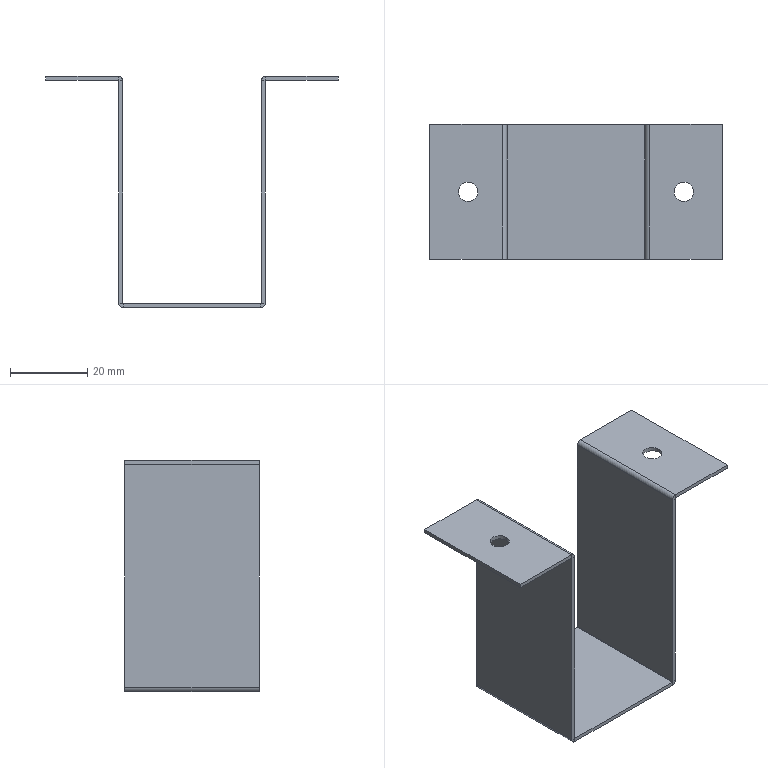Component | SolidWorks | CircuitBreakerBracket_2-1 | 1 solid | 42 faces | box 76 x 35 x 60 mm | volume 6715 mm3 | plane 30 | cylinder 12 | commonest cylinder face diameters 5 x4 2.2 x4 0.2 x4
STEP:
#1=COLOUR_RGB('',0.7922,0.8196,0.9333);
#2=FILL_AREA_STYLE_COLOUR('',#1);
#3=FILL_AREA_STYLE('',(#2));
#4=SURFACE_STYLE_FILL_AREA(#3);
#5=SURFACE_SIDE_STYLE('',(#4));
#6=SURFACE_STYLE_USAGE(.BOTH.,#5);
#7=PRESENTATION_STYLE_ASSIGNMENT((#6));
#8=CARTESIAN_POINT('',(1.068,-1.447,9.771));
#9=VERTEX_POINT('',#8);
#10=CARTESIAN_POINT('',(1.265,-1.447,9.771));
#11=VERTEX_POINT('',#10);
#12=CARTESIAN_POINT('',(1.167,-1.447,9.771));
#13=DIRECTION('',(0.,0.,1.));
#14=DIRECTION('',(1.,0.,0.));
#15=AXIS2_PLACEMENT_3D('',#12,#13,#14);
#16=CIRCLE('',#15,0.09843);
#17=EDGE_CURVE('',#9,#11,#16,.T.);
#18=ORIENTED_EDGE('',*,*,#17,.F.);
#19=CARTESIAN_POINT('',(1.068,-1.447,9.81));
#20=VERTEX_POINT('',#19);
#21=CARTESIAN_POINT('',(1.068,-1.447,9.771));
#22=DIRECTION('',(0.,0.,1.));
#23=VECTOR('',#22,39.37);
#24=LINE('',#21,#23);
#25=EDGE_CURVE('',#9,#20,#24,.T.);
#26=ORIENTED_EDGE('',*,*,#25,.T.);
#27=CARTESIAN_POINT('',(1.265,-1.447,9.81));
#28=VERTEX_POINT('',#27);
#29=CARTESIAN_POINT('',(1.167,-1.447,9.81));
#30=DIRECTION('',(0.,0.,1.));
#31=DIRECTION('',(1.,0.,0.));
#32=AXIS2_PLACEMENT_3D('',#29,#30,#31);
#33=CIRCLE('',#32,0.09843);
#34=EDGE_CURVE('',#20,#28,#33,.T.);
#35=ORIENTED_EDGE('',*,*,#34,.T.);
#36=CARTESIAN_POINT('',(1.265,-1.447,9.771));
#37=DIRECTION('',(0.,0.,1.));
#38=VECTOR('',#37,39.37);
#39=LINE('',#36,#38);
#40=EDGE_CURVE('',#11,#28,#39,.T.);
#41=ORIENTED_EDGE('',*,*,#40,.F.);
#42=EDGE_LOOP('',(#18,#26,#35,#41));
#43=FACE_OUTER_BOUND('',#42,.T.);
#44=CARTESIAN_POINT('',(1.167,-1.447,9.771));
#45=DIRECTION('',(0.,0.,1.));
#46=DIRECTION('',(1.,0.,0.));
#47=AXIS2_PLACEMENT_3D('',#44,#45,#46);
#48=CYLINDRICAL_SURFACE('',#47,0.09843);
#49=ADVANCED_FACE('',(#43),#48,.F.);
#50=CARTESIAN_POINT('',(-1.136,-1.447,9.771));
#51=VERTEX_POINT('',#50);
#52=CARTESIAN_POINT('',(-0.9394,-1.447,9.771));
#53=VERTEX_POINT('',#52);
#54=CARTESIAN_POINT('',(-1.038,-1.447,9.771));
#55=DIRECTION('',(0.,0.,1.));
#56=DIRECTION('',(1.,0.,0.));
#57=AXIS2_PLACEMENT_3D('',#54,#55,#56);
#58=CIRCLE('',#57,0.09843);
#59=EDGE_CURVE('',#51,#53,#58,.T.);
#60=ORIENTED_EDGE('',*,*,#59,.F.);
#61=CARTESIAN_POINT('',(-1.136,-1.447,9.81));
#62=VERTEX_POINT('',#61);
#63=CARTESIAN_POINT('',(-1.136,-1.447,9.771));
#64=DIRECTION('',(0.,0.,1.));
#65=VECTOR('',#64,39.37);
#66=LINE('',#63,#65);
#67=EDGE_CURVE('',#51,#62,#66,.T.);
#68=ORIENTED_EDGE('',*,*,#67,.T.);
#69=CARTESIAN_POINT('',(-0.9394,-1.447,9.81));
#70=VERTEX_POINT('',#69);
#71=CARTESIAN_POINT('',(-1.038,-1.447,9.81));
#72=DIRECTION('',(0.,0.,1.));
#73=DIRECTION('',(1.,0.,0.));
#74=AXIS2_PLACEMENT_3D('',#71,#72,#73);
#75=CIRCLE('',#74,0.09843);
#76=EDGE_CURVE('',#62,#70,#75,.T.);
#77=ORIENTED_EDGE('',*,*,#76,.T.);
#78=CARTESIAN_POINT('',(-0.9394,-1.447,9.771));
#79=DIRECTION('',(0.,0.,1.));
#80=VECTOR('',#79,39.37);
#81=LINE('',#78,#80);
#82=EDGE_CURVE('',#53,#70,#81,.T.);
#83=ORIENTED_EDGE('',*,*,#82,.F.);
#84=EDGE_LOOP('',(#60,#68,#77,#83));
#85=FACE_OUTER_BOUND('',#84,.T.);
#86=CARTESIAN_POINT('',(-1.038,-1.447,9.771));
#87=DIRECTION('',(0.,0.,1.));
#88=DIRECTION('',(1.,0.,0.));
#89=AXIS2_PLACEMENT_3D('',#86,#87,#88);
#90=CYLINDRICAL_SURFACE('',#89,0.09843);
#91=ADVANCED_FACE('',(#85),#90,.F.);
#92=CARTESIAN_POINT('',(0.8126,-2.136,9.767));
#93=VERTEX_POINT('',#92);
#94=CARTESIAN_POINT('',(0.7732,-2.136,9.767));
#95=VERTEX_POINT('',#94);
#96=CARTESIAN_POINT('',(0.8126,-2.136,9.767));
#97=DIRECTION('',(-1.,0.,0.));
#98=VECTOR('',#97,39.37);
#99=LINE('',#96,#98);
#100=EDGE_CURVE('',#93,#95,#99,.T.);
#101=ORIENTED_EDGE('',*,*,#100,.T.);
#102=CARTESIAN_POINT('',(0.7732,-2.136,7.491));
#103=VERTEX_POINT('',#102);
#104=CARTESIAN_POINT('',(0.7732,-2.136,7.488));
#105=DIRECTION('',(-0.,0.,-1.));
#106=VECTOR('',#105,39.37);
#107=LINE('',#104,#106);
#108=EDGE_CURVE('',#95,#103,#107,.T.);
#109=ORIENTED_EDGE('',*,*,#108,.T.);
#110=CARTESIAN_POINT('',(0.8126,-2.136,7.491));
#111=VERTEX_POINT('',#110);
#112=CARTESIAN_POINT('',(0.8126,-2.136,7.491));
#113=DIRECTION('',(1.,0.,-0.));
#114=VECTOR('',#113,39.37);
#115=LINE('',#112,#114);
#116=EDGE_CURVE('',#103,#111,#115,.T.);
#117=ORIENTED_EDGE('',*,*,#116,.T.);
#118=CARTESIAN_POINT('',(0.8126,-2.136,7.488));
#119=DIRECTION('',(-0.,0.,-1.));
#120=VECTOR('',#119,39.37);
#121=LINE('',#118,#120);
#122=EDGE_CURVE('',#93,#111,#121,.T.);
#123=ORIENTED_EDGE('',*,*,#122,.F.);
#124=EDGE_LOOP('',(#101,#109,#117,#123));
#125=FACE_OUTER_BOUND('',#124,.T.);
#126=CARTESIAN_POINT('',(0.8126,-2.136,7.488));
#127=DIRECTION('',(0.,1.,0.));
#128=DIRECTION('',(0.,0.,1.));
#129=AXIS2_PLACEMENT_3D('',#126,#127,#128);
#130=PLANE('',#129);
#131=ADVANCED_FACE('',(#125),#130,.F.);
#132=CARTESIAN_POINT('',(0.8126,-0.7579,9.767));
#133=VERTEX_POINT('',#132);
#134=CARTESIAN_POINT('',(0.7732,-0.7579,9.767));
#135=VERTEX_POINT('',#134);
#136=CARTESIAN_POINT('',(0.8126,-0.7579,9.767));
#137=DIRECTION('',(-1.,0.,0.));
#138=VECTOR('',#137,39.37);
#139=LINE('',#136,#138);
#140=EDGE_CURVE('',#133,#135,#139,.T.);
#141=ORIENTED_EDGE('',*,*,#140,.F.);
#142=CARTESIAN_POINT('',(0.8126,-0.7579,7.491));
#143=VERTEX_POINT('',#142);
#144=CARTESIAN_POINT('',(0.8126,-0.7579,7.488));
#145=DIRECTION('',(0.,0.,1.));
#146=VECTOR('',#145,39.37);
#147=LINE('',#144,#146);
#148=EDGE_CURVE('',#143,#133,#147,.T.);
#149=ORIENTED_EDGE('',*,*,#148,.F.);
#150=CARTESIAN_POINT('',(0.7732,-0.7579,7.491));
#151=VERTEX_POINT('',#150);
#152=CARTESIAN_POINT('',(0.7732,-0.7579,7.491));
#153=DIRECTION('',(1.,0.,-0.));
#154=VECTOR('',#153,39.37);
#155=LINE('',#152,#154);
#156=EDGE_CURVE('',#151,#143,#155,.T.);
#157=ORIENTED_EDGE('',*,*,#156,.F.);
#158=CARTESIAN_POINT('',(0.7732,-0.7579,9.81));
#159=DIRECTION('',(0.,0.,1.));
#160=VECTOR('',#159,39.37);
#161=LINE('',#158,#160);
#162=EDGE_CURVE('',#151,#135,#161,.T.);
#163=ORIENTED_EDGE('',*,*,#162,.T.);
#164=EDGE_LOOP('',(#141,#149,#157,#163));
#165=FACE_OUTER_BOUND('',#164,.T.);
#166=CARTESIAN_POINT('',(0.8126,-0.7579,9.81));
#167=DIRECTION('',(0.,-1.,0.));
#168=DIRECTION('',(0.,0.,-1.));
#169=AXIS2_PLACEMENT_3D('',#166,#167,#168);
#170=PLANE('',#169);
#171=ADVANCED_FACE('',(#165),#170,.F.);
#172=CARTESIAN_POINT('',(0.8126,-2.136,9.767));
#173=DIRECTION('',(0.,1.,0.));
#174=VECTOR('',#173,39.37);
#175=LINE('',#172,#174);
#176=EDGE_CURVE('',#93,#133,#175,.T.);
#177=ORIENTED_EDGE('',*,*,#176,.F.);
#178=ORIENTED_EDGE('',*,*,#122,.T.);
#179=CARTESIAN_POINT('',(0.8126,-2.136,7.491));
#180=DIRECTION('',(-0.,-1.,-0.));
#181=VECTOR('',#180,39.37);
#182=LINE('',#179,#181);
#183=EDGE_CURVE('',#143,#111,#182,.T.);
#184=ORIENTED_EDGE('',*,*,#183,.F.);
#185=ORIENTED_EDGE('',*,*,#148,.T.);
#186=EDGE_LOOP('',(#177,#178,#184,#185));
#187=FACE_OUTER_BOUND('',#186,.T.);
#188=CARTESIAN_POINT('',(0.8126,-2.275,7.488));
#189=DIRECTION('',(-1.,0.,0.));
#190=DIRECTION('',(0.,0.,1.));
#191=AXIS2_PLACEMENT_3D('',#188,#189,#190);
#192=PLANE('',#191);
#193=ADVANCED_FACE('',(#187),#192,.F.);
#194=ORIENTED_EDGE('',*,*,#108,.F.);
#195=CARTESIAN_POINT('',(0.7732,-2.136,9.767));
#196=DIRECTION('',(0.,1.,0.));
#197=VECTOR('',#196,39.37);
#198=LINE('',#195,#197);
#199=EDGE_CURVE('',#95,#135,#198,.T.);
#200=ORIENTED_EDGE('',*,*,#199,.T.);
#201=ORIENTED_EDGE('',*,*,#162,.F.);
#202=CARTESIAN_POINT('',(0.7732,-2.136,7.491));
#203=DIRECTION('',(0.,1.,0.));
#204=VECTOR('',#203,39.37);
#205=LINE('',#202,#204);
#206=EDGE_CURVE('',#103,#151,#205,.T.);
#207=ORIENTED_EDGE('',*,*,#206,.F.);
#208=EDGE_LOOP('',(#194,#200,#201,#207));
#209=FACE_OUTER_BOUND('',#208,.T.);
#210=CARTESIAN_POINT('',(0.7732,-2.275,7.488));
#211=DIRECTION('',(-1.,0.,0.));
#212=DIRECTION('',(0.,0.,1.));
#213=AXIS2_PLACEMENT_3D('',#210,#211,#212);
#214=PLANE('',#213);
#215=ADVANCED_FACE('',(#209),#214,.T.);
#216=CARTESIAN_POINT('',(-0.6835,-0.7579,9.767));
#217=VERTEX_POINT('',#216);
#218=CARTESIAN_POINT('',(-0.6441,-0.7579,9.767));
#219=VERTEX_POINT('',#218);
#220=CARTESIAN_POINT('',(-0.6835,-0.7579,9.767));
#221=DIRECTION('',(1.,0.,0.));
#222=VECTOR('',#221,39.37);
#223=LINE('',#220,#222);
#224=EDGE_CURVE('',#217,#219,#223,.T.);
#225=ORIENTED_EDGE('',*,*,#224,.T.);
#226=CARTESIAN_POINT('',(-0.6441,-0.7579,7.491));
#227=VERTEX_POINT('',#226);
#228=CARTESIAN_POINT('',(-0.6441,-0.7579,7.488));
#229=DIRECTION('',(0.,0.,-1.));
#230=VECTOR('',#229,39.37);
#231=LINE('',#228,#230);
#232=EDGE_CURVE('',#219,#227,#231,.T.);
#233=ORIENTED_EDGE('',*,*,#232,.T.);
#234=CARTESIAN_POINT('',(-0.6835,-0.7579,7.491));
#235=VERTEX_POINT('',#234);
#236=CARTESIAN_POINT('',(-0.6835,-0.7579,7.491));
#237=DIRECTION('',(-1.,0.,-0.));
#238=VECTOR('',#237,39.37);
#239=LINE('',#236,#238);
#240=EDGE_CURVE('',#227,#235,#239,.T.);
#241=ORIENTED_EDGE('',*,*,#240,.T.);
#242=CARTESIAN_POINT('',(-0.6835,-0.7579,7.488));
#243=DIRECTION('',(0.,0.,-1.));
#244=VECTOR('',#243,39.37);
#245=LINE('',#242,#244);
#246=EDGE_CURVE('',#217,#235,#245,.T.);
#247=ORIENTED_EDGE('',*,*,#246,.F.);
#248=EDGE_LOOP('',(#225,#233,#241,#247));
#249=FACE_OUTER_BOUND('',#248,.T.);
#250=CARTESIAN_POINT('',(-0.6835,-0.7579,7.488));
#251=DIRECTION('',(0.,-1.,0.));
#252=DIRECTION('',(0.,0.,-1.));
#253=AXIS2_PLACEMENT_3D('',#250,#251,#252);
#254=PLANE('',#253);
#255=ADVANCED_FACE('',(#249),#254,.F.);
#256=CARTESIAN_POINT('',(-0.6835,-2.136,9.767));
#257=VERTEX_POINT('',#256);
#258=CARTESIAN_POINT('',(-0.6441,-2.136,9.767));
#259=VERTEX_POINT('',#258);
#260=CARTESIAN_POINT('',(-0.6835,-2.136,9.767));
#261=DIRECTION('',(1.,0.,0.));
#262=VECTOR('',#261,39.37);
#263=LINE('',#260,#262);
#264=EDGE_CURVE('',#257,#259,#263,.T.);
#265=ORIENTED_EDGE('',*,*,#264,.F.);
#266=CARTESIAN_POINT('',(-0.6835,-2.136,7.491));
#267=VERTEX_POINT('',#266);
#268=CARTESIAN_POINT('',(-0.6835,-2.136,7.488));
#269=DIRECTION('',(-0.,0.,1.));
#270=VECTOR('',#269,39.37);
#271=LINE('',#268,#270);
#272=EDGE_CURVE('',#267,#257,#271,.T.);
#273=ORIENTED_EDGE('',*,*,#272,.F.);
#274=CARTESIAN_POINT('',(-0.6441,-2.136,7.491));
#275=VERTEX_POINT('',#274);
#276=CARTESIAN_POINT('',(-0.6441,-2.136,7.491));
#277=DIRECTION('',(-1.,0.,-0.));
#278=VECTOR('',#277,39.37);
#279=LINE('',#276,#278);
#280=EDGE_CURVE('',#275,#267,#279,.T.);
#281=ORIENTED_EDGE('',*,*,#280,.F.);
#282=CARTESIAN_POINT('',(-0.6441,-2.136,9.81));
#283=DIRECTION('',(-0.,0.,1.));
#284=VECTOR('',#283,39.37);
#285=LINE('',#282,#284);
#286=EDGE_CURVE('',#275,#259,#285,.T.);
#287=ORIENTED_EDGE('',*,*,#286,.T.);
#288=EDGE_LOOP('',(#265,#273,#281,#287));
#289=FACE_OUTER_BOUND('',#288,.T.);
#290=CARTESIAN_POINT('',(-0.6835,-2.136,9.81));
#291=DIRECTION('',(0.,1.,0.));
#292=DIRECTION('',(0.,0.,1.));
#293=AXIS2_PLACEMENT_3D('',#290,#291,#292);
#294=PLANE('',#293);
#295=ADVANCED_FACE('',(#289),#294,.F.);
#296=CARTESIAN_POINT('',(-0.6835,-0.7579,9.767));
#297=DIRECTION('',(0.,-1.,0.));
#298=VECTOR('',#297,39.37);
#299=LINE('',#296,#298);
#300=EDGE_CURVE('',#217,#257,#299,.T.);
#301=ORIENTED_EDGE('',*,*,#300,.F.);
#302=ORIENTED_EDGE('',*,*,#246,.T.);
#303=CARTESIAN_POINT('',(-0.6835,-0.7579,7.491));
#304=DIRECTION('',(0.,1.,0.));
#305=VECTOR('',#304,39.37);
#306=LINE('',#303,#305);
#307=EDGE_CURVE('',#267,#235,#306,.T.);
#308=ORIENTED_EDGE('',*,*,#307,.F.);
#309=ORIENTED_EDGE('',*,*,#272,.T.);
#310=EDGE_LOOP('',(#301,#302,#308,#309));
#311=FACE_OUTER_BOUND('',#310,.T.);
#312=CARTESIAN_POINT('',(-0.6835,-2.275,7.488));
#313=DIRECTION('',(1.,0.,0.));
#314=DIRECTION('',(0.,0.,-1.));
#315=AXIS2_PLACEMENT_3D('',#312,#313,#314);
#316=PLANE('',#315);
#317=ADVANCED_FACE('',(#311),#316,.F.);
#318=ORIENTED_EDGE('',*,*,#232,.F.);
#319=CARTESIAN_POINT('',(-0.6441,-0.7579,9.767));
#320=DIRECTION('',(0.,-1.,0.));
#321=VECTOR('',#320,39.37);
#322=LINE('',#319,#321);
#323=EDGE_CURVE('',#219,#259,#322,.T.);
#324=ORIENTED_EDGE('',*,*,#323,.T.);
#325=ORIENTED_EDGE('',*,*,#286,.F.);
#326=CARTESIAN_POINT('',(-0.6441,-0.7579,7.491));
#327=DIRECTION('',(0.,-1.,0.));
#328=VECTOR('',#327,39.37);
#329=LINE('',#326,#328);
#330=EDGE_CURVE('',#227,#275,#329,.T.);
#331=ORIENTED_EDGE('',*,*,#330,.F.);
#332=EDGE_LOOP('',(#318,#324,#325,#331));
#333=FACE_OUTER_BOUND('',#332,.T.);
#334=CARTESIAN_POINT('',(-0.6441,-2.275,7.488));
#335=DIRECTION('',(1.,0.,0.));
#336=DIRECTION('',(0.,0.,-1.));
#337=AXIS2_PLACEMENT_3D('',#334,#335,#336);
#338=PLANE('',#337);
#339=ADVANCED_FACE('',(#333),#338,.T.);
#340=CARTESIAN_POINT('',(0.7693,-0.7579,7.448));
#341=VERTEX_POINT('',#340);
#342=CARTESIAN_POINT('',(-0.6402,-0.7579,7.448));
#343=VERTEX_POINT('',#342);
#344=CARTESIAN_POINT('',(-0.6835,-0.7579,7.448));
#345=DIRECTION('',(-1.,0.,0.));
#346=VECTOR('',#345,39.37);
#347=LINE('',#344,#346);
#348=EDGE_CURVE('',#341,#343,#347,.T.);
#349=ORIENTED_EDGE('',*,*,#348,.F.);
#350=CARTESIAN_POINT('',(0.7693,-2.136,7.448));
#351=VERTEX_POINT('',#350);
#352=CARTESIAN_POINT('',(0.7693,-0.7579,7.448));
#353=DIRECTION('',(0.,-1.,0.));
#354=VECTOR('',#353,39.37);
#355=LINE('',#352,#354);
#356=EDGE_CURVE('',#341,#351,#355,.T.);
#357=ORIENTED_EDGE('',*,*,#356,.T.);
#358=CARTESIAN_POINT('',(-0.6402,-2.136,7.448));
#359=VERTEX_POINT('',#358);
#360=CARTESIAN_POINT('',(-0.6835,-2.136,7.448));
#361=DIRECTION('',(1.,0.,0.));
#362=VECTOR('',#361,39.37);
#363=LINE('',#360,#362);
#364=EDGE_CURVE('',#359,#351,#363,.T.);
#365=ORIENTED_EDGE('',*,*,#364,.F.);
#366=CARTESIAN_POINT('',(-0.6402,-2.136,7.448));
#367=DIRECTION('',(0.,1.,0.));
#368=VECTOR('',#367,39.37);
#369=LINE('',#366,#368);
#370=EDGE_CURVE('',#359,#343,#369,.T.);
#371=ORIENTED_EDGE('',*,*,#370,.T.);
#372=EDGE_LOOP('',(#349,#357,#365,#371));
#373=FACE_OUTER_BOUND('',#372,.T.);
#374=CARTESIAN_POINT('',(0.7651,-2.275,7.448));
#375=DIRECTION('',(0.,0.,-1.));
#376=DIRECTION('',(-1.,0.,0.));
#377=AXIS2_PLACEMENT_3D('',#374,#375,#376);
#378=PLANE('',#377);
#379=ADVANCED_FACE('',(#373),#378,.T.);
#380=CARTESIAN_POINT('',(0.7693,-0.7579,7.488));
#381=VERTEX_POINT('',#380);
#382=CARTESIAN_POINT('',(0.7693,-2.136,7.488));
#383=VERTEX_POINT('',#382);
#384=CARTESIAN_POINT('',(0.7693,-0.7579,7.488));
#385=DIRECTION('',(0.,-1.,0.));
#386=VECTOR('',#385,39.37);
#387=LINE('',#384,#386);
#388=EDGE_CURVE('',#381,#383,#387,.T.);
#389=ORIENTED_EDGE('',*,*,#388,.F.);
#390=CARTESIAN_POINT('',(-0.6402,-0.7579,7.488));
#391=VERTEX_POINT('',#390);
#392=CARTESIAN_POINT('',(-0.6835,-0.7579,7.488));
#393=DIRECTION('',(-1.,0.,0.));
#394=VECTOR('',#393,39.37);
#395=LINE('',#392,#394);
#396=EDGE_CURVE('',#381,#391,#395,.T.);
#397=ORIENTED_EDGE('',*,*,#396,.T.);
#398=CARTESIAN_POINT('',(-0.6402,-2.136,7.488));
#399=VERTEX_POINT('',#398);
#400=CARTESIAN_POINT('',(-0.6402,-2.136,7.488));
#401=DIRECTION('',(0.,1.,0.));
#402=VECTOR('',#401,39.37);
#403=LINE('',#400,#402);
#404=EDGE_CURVE('',#399,#391,#403,.T.);
#405=ORIENTED_EDGE('',*,*,#404,.F.);
#406=CARTESIAN_POINT('',(-0.6835,-2.136,7.488));
#407=DIRECTION('',(1.,0.,0.));
#408=VECTOR('',#407,39.37);
#409=LINE('',#406,#408);
#410=EDGE_CURVE('',#399,#383,#409,.T.);
#411=ORIENTED_EDGE('',*,*,#410,.T.);
#412=EDGE_LOOP('',(#389,#397,#405,#411));
#413=FACE_OUTER_BOUND('',#412,.T.);
#414=CARTESIAN_POINT('',(0.7651,-2.275,7.488));
#415=DIRECTION('',(0.,0.,-1.));
#416=DIRECTION('',(-1.,0.,0.));
#417=AXIS2_PLACEMENT_3D('',#414,#415,#416);
#418=PLANE('',#417);
#419=ADVANCED_FACE('',(#413),#418,.F.);
#420=ORIENTED_EDGE('',*,*,#396,.F.);
#421=CARTESIAN_POINT('',(0.7693,-0.7579,7.488));
#422=DIRECTION('',(0.,0.,-1.));
#423=VECTOR('',#422,39.37);
#424=LINE('',#421,#423);
#425=EDGE_CURVE('',#381,#341,#424,.T.);
#426=ORIENTED_EDGE('',*,*,#425,.T.);
#427=ORIENTED_EDGE('',*,*,#348,.T.);
#428=CARTESIAN_POINT('',(-0.6402,-0.7579,7.488));
#429=DIRECTION('',(0.,0.,-1.));
#430=VECTOR('',#429,39.37);
#431=LINE('',#428,#430);
#432=EDGE_CURVE('',#391,#343,#431,.T.);
#433=ORIENTED_EDGE('',*,*,#432,.F.);
#434=EDGE_LOOP('',(#420,#426,#427,#433));
#435=FACE_OUTER_BOUND('',#434,.T.);
#436=CARTESIAN_POINT('',(-0.6835,-0.7579,7.448));
#437=DIRECTION('',(0.,1.,0.));
#438=DIRECTION('',(0.,0.,1.));
#439=AXIS2_PLACEMENT_3D('',#436,#437,#438);
#440=PLANE('',#439);
#441=ADVANCED_FACE('',(#435),#440,.T.);
#442=CARTESIAN_POINT('',(0.7693,-2.136,7.488));
#443=DIRECTION('',(0.,0.,-1.));
#444=VECTOR('',#443,39.37);
#445=LINE('',#442,#444);
#446=EDGE_CURVE('',#383,#351,#445,.T.);
#447=ORIENTED_EDGE('',*,*,#446,.F.);
#448=ORIENTED_EDGE('',*,*,#410,.F.);
#449=CARTESIAN_POINT('',(-0.6402,-2.136,7.488));
#450=DIRECTION('',(0.,0.,-1.));
#451=VECTOR('',#450,39.37);
#452=LINE('',#449,#451);
#453=EDGE_CURVE('',#399,#359,#452,.T.);
#454=ORIENTED_EDGE('',*,*,#453,.T.);
#455=ORIENTED_EDGE('',*,*,#364,.T.);
#456=EDGE_LOOP('',(#447,#448,#454,#455));
#457=FACE_OUTER_BOUND('',#456,.T.);
#458=CARTESIAN_POINT('',(-0.6835,-2.136,7.448));
#459=DIRECTION('',(0.,-1.,0.));
#460=DIRECTION('',(0.,0.,-1.));
#461=AXIS2_PLACEMENT_3D('',#458,#459,#460);
#462=PLANE('',#461);
#463=ADVANCED_FACE('',(#457),#462,.T.);
#464=ORIENTED_EDGE('',*,*,#240,.F.);
#465=CARTESIAN_POINT('',(-0.6402,-0.7579,7.491));
#466=DIRECTION('',(0.,1.,0.));
#467=DIRECTION('',(0.,0.,-1.));
#468=AXIS2_PLACEMENT_3D('',#465,#466,#467);
#469=CIRCLE('',#468,0.003937);
#470=EDGE_CURVE('',#391,#227,#469,.T.);
#471=ORIENTED_EDGE('',*,*,#470,.F.);
#472=ORIENTED_EDGE('',*,*,#432,.T.);
#473=CARTESIAN_POINT('',(-0.6402,-0.7579,7.491));
#474=DIRECTION('',(0.,1.,0.));
#475=DIRECTION('',(0.,0.,-1.));
#476=AXIS2_PLACEMENT_3D('',#473,#474,#475);
#477=CIRCLE('',#476,0.04331);
#478=EDGE_CURVE('',#343,#235,#477,.T.);
#479=ORIENTED_EDGE('',*,*,#478,.T.);
#480=EDGE_LOOP('',(#464,#471,#472,#479));
#481=FACE_OUTER_BOUND('',#480,.T.);
#482=CARTESIAN_POINT('',(-0.6402,-0.7579,7.491));
#483=DIRECTION('',(0.,1.,0.));
#484=DIRECTION('',(0.,0.,1.));
#485=AXIS2_PLACEMENT_3D('',#482,#483,#484);
#486=PLANE('',#485);
#487=ADVANCED_FACE('',(#481),#486,.T.);
#488=CARTESIAN_POINT('',(-0.6402,-2.136,7.491));
#489=DIRECTION('',(0.,-1.,0.));
#490=DIRECTION('',(0.,0.,-1.));
#491=AXIS2_PLACEMENT_3D('',#488,#489,#490);
#492=CIRCLE('',#491,0.003937);
#493=EDGE_CURVE('',#275,#399,#492,.T.);
#494=ORIENTED_EDGE('',*,*,#493,.F.);
#495=ORIENTED_EDGE('',*,*,#280,.T.);
#496=CARTESIAN_POINT('',(-0.6402,-2.136,7.491));
#497=DIRECTION('',(0.,-1.,0.));
#498=DIRECTION('',(0.,0.,-1.));
#499=AXIS2_PLACEMENT_3D('',#496,#497,#498);
#500=CIRCLE('',#499,0.04331);
#501=EDGE_CURVE('',#267,#359,#500,.T.);
#502=ORIENTED_EDGE('',*,*,#501,.T.);
#503=ORIENTED_EDGE('',*,*,#453,.F.);
#504=EDGE_LOOP('',(#494,#495,#502,#503));
#505=FACE_OUTER_BOUND('',#504,.T.);
#506=CARTESIAN_POINT('',(-0.6402,-2.136,7.491));
#507=DIRECTION('',(0.,1.,0.));
#508=DIRECTION('',(0.,0.,1.));
#509=AXIS2_PLACEMENT_3D('',#506,#507,#508);
#510=PLANE('',#509);
#511=ADVANCED_FACE('',(#505),#510,.F.);
#512=ORIENTED_EDGE('',*,*,#370,.F.);
#513=ORIENTED_EDGE('',*,*,#501,.F.);
#514=ORIENTED_EDGE('',*,*,#307,.T.);
#515=ORIENTED_EDGE('',*,*,#478,.F.);
#516=EDGE_LOOP('',(#512,#513,#514,#515));
#517=FACE_OUTER_BOUND('',#516,.T.);
#518=CARTESIAN_POINT('',(-0.6402,-2.136,7.491));
#519=DIRECTION('',(0.,-1.,0.));
#520=DIRECTION('',(-1.,0.,0.));
#521=AXIS2_PLACEMENT_3D('',#518,#519,#520);
#522=CYLINDRICAL_SURFACE('',#521,0.04331);
#523=ADVANCED_FACE('',(#517),#522,.T.);
#524=ORIENTED_EDGE('',*,*,#404,.T.);
#525=ORIENTED_EDGE('',*,*,#470,.T.);
#526=ORIENTED_EDGE('',*,*,#330,.T.);
#527=ORIENTED_EDGE('',*,*,#493,.T.);
#528=EDGE_LOOP('',(#524,#525,#526,#527));
#529=FACE_OUTER_BOUND('',#528,.T.);
#530=CARTESIAN_POINT('',(-0.6402,-2.136,7.491));
#531=DIRECTION('',(0.,-1.,0.));
#532=DIRECTION('',(-1.,0.,0.));
#533=AXIS2_PLACEMENT_3D('',#530,#531,#532);
#534=CYLINDRICAL_SURFACE('',#533,0.003937);
#535=ADVANCED_FACE('',(#529),#534,.F.);
#536=ORIENTED_EDGE('',*,*,#116,.F.);
#537=CARTESIAN_POINT('',(0.7693,-2.136,7.491));
#538=DIRECTION('',(0.,-1.,0.));
#539=DIRECTION('',(-1.,0.,0.));
#540=AXIS2_PLACEMENT_3D('',#537,#538,#539);
#541=CIRCLE('',#540,0.003937);
#542=EDGE_CURVE('',#383,#103,#541,.T.);
#543=ORIENTED_EDGE('',*,*,#542,.F.);
#544=ORIENTED_EDGE('',*,*,#446,.T.);
#545=CARTESIAN_POINT('',(0.7693,-2.136,7.491));
#546=DIRECTION('',(0.,-1.,0.));
#547=DIRECTION('',(-1.,0.,0.));
#548=AXIS2_PLACEMENT_3D('',#545,#546,#547);
#549=CIRCLE('',#548,0.04331);
#550=EDGE_CURVE('',#351,#111,#549,.T.);
#551=ORIENTED_EDGE('',*,*,#550,.T.);
#552=EDGE_LOOP('',(#536,#543,#544,#551));
#553=FACE_OUTER_BOUND('',#552,.T.);
#554=CARTESIAN_POINT('',(0.7693,-2.136,7.491));
#555=DIRECTION('',(0.,-1.,0.));
#556=DIRECTION('',(1.,0.,0.));
#557=AXIS2_PLACEMENT_3D('',#554,#555,#556);
#558=PLANE('',#557);
#559=ADVANCED_FACE('',(#553),#558,.T.);
#560=CARTESIAN_POINT('',(0.7693,-0.7579,7.491));
#561=DIRECTION('',(-0.,1.,0.));
#562=DIRECTION('',(-1.,0.,0.));
#563=AXIS2_PLACEMENT_3D('',#560,#561,#562);
#564=CIRCLE('',#563,0.003937);
#565=EDGE_CURVE('',#151,#381,#564,.T.);
#566=ORIENTED_EDGE('',*,*,#565,.F.);
#567=ORIENTED_EDGE('',*,*,#156,.T.);
#568=CARTESIAN_POINT('',(0.7693,-0.7579,7.491));
#569=DIRECTION('',(-0.,1.,0.));
#570=DIRECTION('',(-1.,0.,0.));
#571=AXIS2_PLACEMENT_3D('',#568,#569,#570);
#572=CIRCLE('',#571,0.04331);
#573=EDGE_CURVE('',#143,#341,#572,.T.);
#574=ORIENTED_EDGE('',*,*,#573,.T.);
#575=ORIENTED_EDGE('',*,*,#425,.F.);
#576=EDGE_LOOP('',(#566,#567,#574,#575));
#577=FACE_OUTER_BOUND('',#576,.T.);
#578=CARTESIAN_POINT('',(0.7693,-0.7579,7.491));
#579=DIRECTION('',(0.,-1.,0.));
#580=DIRECTION('',(1.,0.,0.));
#581=AXIS2_PLACEMENT_3D('',#578,#579,#580);
#582=PLANE('',#581);
#583=ADVANCED_FACE('',(#577),#582,.F.);
#584=ORIENTED_EDGE('',*,*,#356,.F.);
#585=ORIENTED_EDGE('',*,*,#573,.F.);
#586=ORIENTED_EDGE('',*,*,#183,.T.);
#587=ORIENTED_EDGE('',*,*,#550,.F.);
#588=EDGE_LOOP('',(#584,#585,#586,#587));
#589=FACE_OUTER_BOUND('',#588,.T.);
#590=CARTESIAN_POINT('',(0.7693,-0.7579,7.491));
#591=DIRECTION('',(-0.,1.,0.));
#592=DIRECTION('',(1.,0.,0.));
#593=AXIS2_PLACEMENT_3D('',#590,#591,#592);
#594=CYLINDRICAL_SURFACE('',#593,0.04331);
#595=ADVANCED_FACE('',(#589),#594,.T.);
#596=ORIENTED_EDGE('',*,*,#388,.T.);
#597=ORIENTED_EDGE('',*,*,#542,.T.);
#598=ORIENTED_EDGE('',*,*,#206,.T.);
#599=ORIENTED_EDGE('',*,*,#565,.T.);
#600=EDGE_LOOP('',(#596,#597,#598,#599));
#601=FACE_OUTER_BOUND('',#600,.T.);
#602=CARTESIAN_POINT('',(0.7693,-0.7579,7.491));
#603=DIRECTION('',(-0.,1.,0.));
#604=DIRECTION('',(1.,0.,0.));
#605=AXIS2_PLACEMENT_3D('',#602,#603,#604);
#606=CYLINDRICAL_SURFACE('',#605,0.003937);
#607=ADVANCED_FACE('',(#601),#606,.F.);
#608=CARTESIAN_POINT('',(-0.6874,-2.136,9.771));
#609=VERTEX_POINT('',#608);
#610=CARTESIAN_POINT('',(-0.6874,-2.136,9.81));
#611=VERTEX_POINT('',#610);
#612=CARTESIAN_POINT('',(-0.6874,-2.136,9.81));
#613=DIRECTION('',(0.,0.,1.));
#614=VECTOR('',#613,39.37);
#615=LINE('',#612,#614);
#616=EDGE_CURVE('',#609,#611,#615,.T.);
#617=ORIENTED_EDGE('',*,*,#616,.F.);
#618=CARTESIAN_POINT('',(-0.6874,-2.136,9.767));
#619=DIRECTION('',(0.,-1.,0.));
#620=DIRECTION('',(0.,0.,1.));
#621=AXIS2_PLACEMENT_3D('',#618,#619,#620);
#622=CIRCLE('',#621,0.003937);
#623=EDGE_CURVE('',#257,#609,#622,.T.);
#624=ORIENTED_EDGE('',*,*,#623,.F.);
#625=ORIENTED_EDGE('',*,*,#264,.T.);
#626=CARTESIAN_POINT('',(-0.6874,-2.136,9.767));
#627=DIRECTION('',(0.,-1.,0.));
#628=DIRECTION('',(0.,0.,1.));
#629=AXIS2_PLACEMENT_3D('',#626,#627,#628);
#630=CIRCLE('',#629,0.04331);
#631=EDGE_CURVE('',#259,#611,#630,.T.);
#632=ORIENTED_EDGE('',*,*,#631,.T.);
#633=EDGE_LOOP('',(#617,#624,#625,#632));
#634=FACE_OUTER_BOUND('',#633,.T.);
#635=CARTESIAN_POINT('',(-0.6874,-2.136,9.767));
#636=DIRECTION('',(0.,-1.,0.));
#637=DIRECTION('',(0.,0.,-1.));
#638=AXIS2_PLACEMENT_3D('',#635,#636,#637);
#639=PLANE('',#638);
#640=ADVANCED_FACE('',(#634),#639,.T.);
#641=CARTESIAN_POINT('',(-0.6874,-0.7579,9.771));
#642=VERTEX_POINT('',#641);
#643=CARTESIAN_POINT('',(-0.6874,-0.7579,9.767));
#644=DIRECTION('',(0.,1.,0.));
#645=DIRECTION('',(0.,0.,1.));
#646=AXIS2_PLACEMENT_3D('',#643,#644,#645);
#647=CIRCLE('',#646,0.003937);
#648=EDGE_CURVE('',#642,#217,#647,.T.);
#649=ORIENTED_EDGE('',*,*,#648,.F.);
#650=CARTESIAN_POINT('',(-0.6874,-0.7579,9.81));
#651=VERTEX_POINT('',#650);
#652=CARTESIAN_POINT('',(-0.6874,-0.7579,9.771));
#653=DIRECTION('',(0.,0.,1.));
#654=VECTOR('',#653,39.37);
#655=LINE('',#652,#654);
#656=EDGE_CURVE('',#642,#651,#655,.T.);
#657=ORIENTED_EDGE('',*,*,#656,.T.);
#658=CARTESIAN_POINT('',(-0.6874,-0.7579,9.767));
#659=DIRECTION('',(0.,1.,0.));
#660=DIRECTION('',(0.,0.,1.));
#661=AXIS2_PLACEMENT_3D('',#658,#659,#660);
#662=CIRCLE('',#661,0.04331);
#663=EDGE_CURVE('',#651,#219,#662,.T.);
#664=ORIENTED_EDGE('',*,*,#663,.T.);
#665=ORIENTED_EDGE('',*,*,#224,.F.);
#666=EDGE_LOOP('',(#649,#657,#664,#665));
#667=FACE_OUTER_BOUND('',#666,.T.);
#668=CARTESIAN_POINT('',(-0.6874,-0.7579,9.767));
#669=DIRECTION('',(0.,-1.,0.));
#670=DIRECTION('',(0.,0.,-1.));
#671=AXIS2_PLACEMENT_3D('',#668,#669,#670);
#672=PLANE('',#671);
#673=ADVANCED_FACE('',(#667),#672,.F.);
#674=ORIENTED_EDGE('',*,*,#323,.F.);
#675=ORIENTED_EDGE('',*,*,#663,.F.);
#676=CARTESIAN_POINT('',(-0.6874,-2.275,9.81));
#677=DIRECTION('',(0.,1.,0.));
#678=VECTOR('',#677,39.37);
#679=LINE('',#676,#678);
#680=EDGE_CURVE('',#611,#651,#679,.T.);
#681=ORIENTED_EDGE('',*,*,#680,.F.);
#682=ORIENTED_EDGE('',*,*,#631,.F.);
#683=EDGE_LOOP('',(#674,#675,#681,#682));
#684=FACE_OUTER_BOUND('',#683,.T.);
#685=CARTESIAN_POINT('',(-0.6874,-0.7579,9.767));
#686=DIRECTION('',(0.,1.,0.));
#687=DIRECTION('',(0.,0.,1.));
#688=AXIS2_PLACEMENT_3D('',#685,#686,#687);
#689=CYLINDRICAL_SURFACE('',#688,0.04331);
#690=ADVANCED_FACE('',(#684),#689,.T.);
#691=ORIENTED_EDGE('',*,*,#300,.T.);
#692=ORIENTED_EDGE('',*,*,#623,.T.);
#693=CARTESIAN_POINT('',(-0.6874,-2.136,9.771));
#694=DIRECTION('',(0.,1.,0.));
#695=VECTOR('',#694,39.37);
#696=LINE('',#693,#695);
#697=EDGE_CURVE('',#609,#642,#696,.T.);
#698=ORIENTED_EDGE('',*,*,#697,.T.);
#699=ORIENTED_EDGE('',*,*,#648,.T.);
#700=EDGE_LOOP('',(#691,#692,#698,#699));
#701=FACE_OUTER_BOUND('',#700,.T.);
#702=CARTESIAN_POINT('',(-0.6874,-0.7579,9.767));
#703=DIRECTION('',(0.,1.,0.));
#704=DIRECTION('',(0.,0.,1.));
#705=AXIS2_PLACEMENT_3D('',#702,#703,#704);
#706=CYLINDRICAL_SURFACE('',#705,0.003937);
#707=ADVANCED_FACE('',(#701),#706,.F.);
#708=CARTESIAN_POINT('',(-1.432,-0.7579,9.81));
#709=VERTEX_POINT('',#708);
#710=CARTESIAN_POINT('',(-0.6835,-0.7579,9.81));
#711=DIRECTION('',(1.,0.,0.));
#712=VECTOR('',#711,39.37);
#713=LINE('',#710,#712);
#714=EDGE_CURVE('',#709,#651,#713,.T.);
#715=ORIENTED_EDGE('',*,*,#714,.T.);
#716=ORIENTED_EDGE('',*,*,#656,.F.);
#717=CARTESIAN_POINT('',(-1.432,-0.7579,9.771));
#718=VERTEX_POINT('',#717);
#719=CARTESIAN_POINT('',(0.7651,-0.7579,9.771));
#720=DIRECTION('',(1.,0.,0.));
#721=VECTOR('',#720,39.37);
#722=LINE('',#719,#721);
#723=EDGE_CURVE('',#718,#642,#722,.T.);
#724=ORIENTED_EDGE('',*,*,#723,.F.);
#725=CARTESIAN_POINT('',(-1.432,-0.7579,9.81));
#726=DIRECTION('',(0.,0.,-1.));
#727=VECTOR('',#726,39.37);
#728=LINE('',#725,#727);
#729=EDGE_CURVE('',#709,#718,#728,.T.);
#730=ORIENTED_EDGE('',*,*,#729,.F.);
#731=EDGE_LOOP('',(#715,#716,#724,#730));
#732=FACE_OUTER_BOUND('',#731,.T.);
#733=CARTESIAN_POINT('',(-0.6835,-0.7579,9.81));
#734=DIRECTION('',(0.,1.,0.));
#735=DIRECTION('',(0.,0.,1.));
#736=AXIS2_PLACEMENT_3D('',#733,#734,#735);
#737=PLANE('',#736);
#738=ADVANCED_FACE('',(#732),#737,.T.);
#739=CARTESIAN_POINT('',(-1.432,-2.136,9.771));
#740=VERTEX_POINT('',#739);
#741=CARTESIAN_POINT('',(0.7651,-2.136,9.771));
#742=DIRECTION('',(-1.,0.,0.));
#743=VECTOR('',#742,39.37);
#744=LINE('',#741,#743);
#745=EDGE_CURVE('',#609,#740,#744,.T.);
#746=ORIENTED_EDGE('',*,*,#745,.F.);
#747=ORIENTED_EDGE('',*,*,#616,.T.);
#748=CARTESIAN_POINT('',(-1.432,-2.136,9.81));
#749=VERTEX_POINT('',#748);
#750=CARTESIAN_POINT('',(-1.432,-2.136,9.81));
#751=DIRECTION('',(-1.,0.,0.));
#752=VECTOR('',#751,39.37);
#753=LINE('',#750,#752);
#754=EDGE_CURVE('',#611,#749,#753,.T.);
#755=ORIENTED_EDGE('',*,*,#754,.T.);
#756=CARTESIAN_POINT('',(-1.432,-2.136,9.81));
#757=DIRECTION('',(0.,0.,-1.));
#758=VECTOR('',#757,39.37);
#759=LINE('',#756,#758);
#760=EDGE_CURVE('',#749,#740,#759,.T.);
#761=ORIENTED_EDGE('',*,*,#760,.T.);
#762=EDGE_LOOP('',(#746,#747,#755,#761));
#763=FACE_OUTER_BOUND('',#762,.T.);
#764=CARTESIAN_POINT('',(-1.432,-2.136,9.81));
#765=DIRECTION('',(0.,-1.,0.));
#766=DIRECTION('',(0.,0.,-1.));
#767=AXIS2_PLACEMENT_3D('',#764,#765,#766);
#768=PLANE('',#767);
#769=ADVANCED_FACE('',(#763),#768,.T.);
#770=CARTESIAN_POINT('',(-1.038,-1.447,9.81));
#771=DIRECTION('',(0.,0.,1.));
#772=DIRECTION('',(1.,0.,0.));
#773=AXIS2_PLACEMENT_3D('',#770,#771,#772);
#774=CIRCLE('',#773,0.09843);
#775=EDGE_CURVE('',#70,#62,#774,.T.);
#776=ORIENTED_EDGE('',*,*,#775,.F.);
#777=ORIENTED_EDGE('',*,*,#76,.F.);
#778=EDGE_LOOP('',(#776,#777));
#779=FACE_BOUND('',#778,.T.);
#780=ORIENTED_EDGE('',*,*,#754,.F.);
#781=ORIENTED_EDGE('',*,*,#680,.T.);
#782=ORIENTED_EDGE('',*,*,#714,.F.);
#783=CARTESIAN_POINT('',(-1.432,-0.7579,9.81));
#784=DIRECTION('',(0.,1.,0.));
#785=VECTOR('',#784,39.37);
#786=LINE('',#783,#785);
#787=EDGE_CURVE('',#749,#709,#786,.T.);
#788=ORIENTED_EDGE('',*,*,#787,.F.);
#789=EDGE_LOOP('',(#780,#781,#782,#788));
#790=FACE_OUTER_BOUND('',#789,.T.);
#791=CARTESIAN_POINT('',(0.7651,-2.275,9.81));
#792=DIRECTION('',(0.,0.,1.));
#793=DIRECTION('',(1.,0.,0.));
#794=AXIS2_PLACEMENT_3D('',#791,#792,#793);
#795=PLANE('',#794);
#796=ADVANCED_FACE('',(#779,#790),#795,.T.);
#797=CARTESIAN_POINT('',(-1.038,-1.447,9.771));
#798=DIRECTION('',(0.,0.,1.));
#799=DIRECTION('',(1.,0.,0.));
#800=AXIS2_PLACEMENT_3D('',#797,#798,#799);
#801=CIRCLE('',#800,0.09843);
#802=EDGE_CURVE('',#53,#51,#801,.T.);
#803=ORIENTED_EDGE('',*,*,#802,.T.);
#804=ORIENTED_EDGE('',*,*,#59,.T.);
#805=EDGE_LOOP('',(#803,#804));
#806=FACE_BOUND('',#805,.T.);
#807=ORIENTED_EDGE('',*,*,#697,.F.);
#808=ORIENTED_EDGE('',*,*,#745,.T.);
#809=CARTESIAN_POINT('',(-1.432,-2.275,9.771));
#810=DIRECTION('',(0.,1.,0.));
#811=VECTOR('',#810,39.37);
#812=LINE('',#809,#811);
#813=EDGE_CURVE('',#740,#718,#812,.T.);
#814=ORIENTED_EDGE('',*,*,#813,.T.);
#815=ORIENTED_EDGE('',*,*,#723,.T.);
#816=EDGE_LOOP('',(#807,#808,#814,#815));
#817=FACE_OUTER_BOUND('',#816,.T.);
#818=CARTESIAN_POINT('',(0.7651,-2.275,9.771));
#819=DIRECTION('',(0.,0.,1.));
#820=DIRECTION('',(1.,0.,0.));
#821=AXIS2_PLACEMENT_3D('',#818,#819,#820);
#822=PLANE('',#821);
#823=ADVANCED_FACE('',(#806,#817),#822,.F.);
#824=ORIENTED_EDGE('',*,*,#813,.F.);
#825=ORIENTED_EDGE('',*,*,#760,.F.);
#826=ORIENTED_EDGE('',*,*,#787,.T.);
#827=ORIENTED_EDGE('',*,*,#729,.T.);
#828=EDGE_LOOP('',(#824,#825,#826,#827));
#829=FACE_OUTER_BOUND('',#828,.T.);
#830=CARTESIAN_POINT('',(-1.432,-0.7579,9.81));
#831=DIRECTION('',(-1.,0.,-0.));
#832=DIRECTION('',(-0.,0.,1.));
#833=AXIS2_PLACEMENT_3D('',#830,#831,#832);
#834=PLANE('',#833);
#835=ADVANCED_FACE('',(#829),#834,.T.);
#836=CARTESIAN_POINT('',(0.8165,-0.7579,9.771));
#837=VERTEX_POINT('',#836);
#838=CARTESIAN_POINT('',(0.8165,-0.7579,9.81));
#839=VERTEX_POINT('',#838);
#840=CARTESIAN_POINT('',(0.8165,-0.7579,9.81));
#841=DIRECTION('',(0.,0.,1.));
#842=VECTOR('',#841,39.37);
#843=LINE('',#840,#842);
#844=EDGE_CURVE('',#837,#839,#843,.T.);
#845=ORIENTED_EDGE('',*,*,#844,.F.);
#846=CARTESIAN_POINT('',(0.8165,-0.7579,9.767));
#847=DIRECTION('',(0.,1.,0.));
#848=DIRECTION('',(0.,0.,-1.));
#849=AXIS2_PLACEMENT_3D('',#846,#847,#848);
#850=CIRCLE('',#849,0.003937);
#851=EDGE_CURVE('',#133,#837,#850,.T.);
#852=ORIENTED_EDGE('',*,*,#851,.F.);
#853=ORIENTED_EDGE('',*,*,#140,.T.);
#854=CARTESIAN_POINT('',(0.8165,-0.7579,9.767));
#855=DIRECTION('',(0.,1.,0.));
#856=DIRECTION('',(0.,0.,-1.));
#857=AXIS2_PLACEMENT_3D('',#854,#855,#856);
#858=CIRCLE('',#857,0.04331);
#859=EDGE_CURVE('',#135,#839,#858,.T.);
#860=ORIENTED_EDGE('',*,*,#859,.T.);
#861=EDGE_LOOP('',(#845,#852,#853,#860));
#862=FACE_OUTER_BOUND('',#861,.T.);
#863=CARTESIAN_POINT('',(0.8165,-0.7579,9.767));
#864=DIRECTION('',(0.,1.,0.));
#865=DIRECTION('',(0.,0.,1.));
#866=AXIS2_PLACEMENT_3D('',#863,#864,#865);
#867=PLANE('',#866);
#868=ADVANCED_FACE('',(#862),#867,.T.);
#869=CARTESIAN_POINT('',(0.8165,-2.136,9.771));
#870=VERTEX_POINT('',#869);
#871=CARTESIAN_POINT('',(0.8165,-2.136,9.767));
#872=DIRECTION('',(0.,-1.,0.));
#873=DIRECTION('',(0.,0.,-1.));
#874=AXIS2_PLACEMENT_3D('',#871,#872,#873);
#875=CIRCLE('',#874,0.003937);
#876=EDGE_CURVE('',#870,#93,#875,.T.);
#877=ORIENTED_EDGE('',*,*,#876,.F.);
#878=CARTESIAN_POINT('',(0.8165,-2.136,9.81));
#879=VERTEX_POINT('',#878);
#880=CARTESIAN_POINT('',(0.8165,-2.136,9.771));
#881=DIRECTION('',(0.,0.,1.));
#882=VECTOR('',#881,39.37);
#883=LINE('',#880,#882);
#884=EDGE_CURVE('',#870,#879,#883,.T.);
#885=ORIENTED_EDGE('',*,*,#884,.T.);
#886=CARTESIAN_POINT('',(0.8165,-2.136,9.767));
#887=DIRECTION('',(0.,-1.,0.));
#888=DIRECTION('',(0.,0.,-1.));
#889=AXIS2_PLACEMENT_3D('',#886,#887,#888);
#890=CIRCLE('',#889,0.04331);
#891=EDGE_CURVE('',#879,#95,#890,.T.);
#892=ORIENTED_EDGE('',*,*,#891,.T.);
#893=ORIENTED_EDGE('',*,*,#100,.F.);
#894=EDGE_LOOP('',(#877,#885,#892,#893));
#895=FACE_OUTER_BOUND('',#894,.T.);
#896=CARTESIAN_POINT('',(0.8165,-2.136,9.767));
#897=DIRECTION('',(0.,1.,0.));
#898=DIRECTION('',(0.,0.,1.));
#899=AXIS2_PLACEMENT_3D('',#896,#897,#898);
#900=PLANE('',#899);
#901=ADVANCED_FACE('',(#895),#900,.F.);
#902=ORIENTED_EDGE('',*,*,#199,.F.);
#903=ORIENTED_EDGE('',*,*,#891,.F.);
#904=CARTESIAN_POINT('',(0.8165,-0.7579,9.81));
#905=DIRECTION('',(0.,1.,0.));
#906=VECTOR('',#905,39.37);
#907=LINE('',#904,#906);
#908=EDGE_CURVE('',#879,#839,#907,.T.);
#909=ORIENTED_EDGE('',*,*,#908,.T.);
#910=ORIENTED_EDGE('',*,*,#859,.F.);
#911=EDGE_LOOP('',(#902,#903,#909,#910));
#912=FACE_OUTER_BOUND('',#911,.T.);
#913=CARTESIAN_POINT('',(0.8165,-2.136,9.767));
#914=DIRECTION('',(0.,-1.,0.));
#915=DIRECTION('',(0.,0.,1.));
#916=AXIS2_PLACEMENT_3D('',#913,#914,#915);
#917=CYLINDRICAL_SURFACE('',#916,0.04331);
#918=ADVANCED_FACE('',(#912),#917,.T.);
#919=ORIENTED_EDGE('',*,*,#176,.T.);
#920=ORIENTED_EDGE('',*,*,#851,.T.);
#921=CARTESIAN_POINT('',(0.8165,-0.7579,9.771));
#922=DIRECTION('',(0.,-1.,0.));
#923=VECTOR('',#922,39.37);
#924=LINE('',#921,#923);
#925=EDGE_CURVE('',#837,#870,#924,.T.);
#926=ORIENTED_EDGE('',*,*,#925,.T.);
#927=ORIENTED_EDGE('',*,*,#876,.T.);
#928=EDGE_LOOP('',(#919,#920,#926,#927));
#929=FACE_OUTER_BOUND('',#928,.T.);
#930=CARTESIAN_POINT('',(0.8165,-2.136,9.767));
#931=DIRECTION('',(0.,-1.,0.));
#932=DIRECTION('',(0.,0.,1.));
#933=AXIS2_PLACEMENT_3D('',#930,#931,#932);
#934=CYLINDRICAL_SURFACE('',#933,0.003937);
#935=ADVANCED_FACE('',(#929),#934,.F.);
#936=CARTESIAN_POINT('',(1.561,-0.7579,9.771));
#937=VERTEX_POINT('',#936);
#938=CARTESIAN_POINT('',(0.7651,-0.7579,9.771));
#939=DIRECTION('',(1.,0.,0.));
#940=VECTOR('',#939,39.37);
#941=LINE('',#938,#940);
#942=EDGE_CURVE('',#837,#937,#941,.T.);
#943=ORIENTED_EDGE('',*,*,#942,.F.);
#944=ORIENTED_EDGE('',*,*,#844,.T.);
#945=CARTESIAN_POINT('',(1.561,-0.7579,9.81));
#946=VERTEX_POINT('',#945);
#947=CARTESIAN_POINT('',(0.8126,-0.7579,9.81));
#948=DIRECTION('',(1.,0.,0.));
#949=VECTOR('',#948,39.37);
#950=LINE('',#947,#949);
#951=EDGE_CURVE('',#839,#946,#950,.T.);
#952=ORIENTED_EDGE('',*,*,#951,.T.);
#953=CARTESIAN_POINT('',(1.561,-0.7579,9.81));
#954=DIRECTION('',(-0.,0.,-1.));
#955=VECTOR('',#954,39.37);
#956=LINE('',#953,#955);
#957=EDGE_CURVE('',#946,#937,#956,.T.);
#958=ORIENTED_EDGE('',*,*,#957,.T.);
#959=EDGE_LOOP('',(#943,#944,#952,#958));
#960=FACE_OUTER_BOUND('',#959,.T.);
#961=CARTESIAN_POINT('',(0.8126,-0.7579,9.81));
#962=DIRECTION('',(0.,1.,0.));
#963=DIRECTION('',(0.,0.,1.));
#964=AXIS2_PLACEMENT_3D('',#961,#962,#963);
#965=PLANE('',#964);
#966=ADVANCED_FACE('',(#960),#965,.T.);
#967=CARTESIAN_POINT('',(1.561,-2.136,9.81));
#968=VERTEX_POINT('',#967);
#969=CARTESIAN_POINT('',(1.561,-2.136,9.81));
#970=DIRECTION('',(-1.,0.,0.));
#971=VECTOR('',#970,39.37);
#972=LINE('',#969,#971);
#973=EDGE_CURVE('',#968,#879,#972,.T.);
#974=ORIENTED_EDGE('',*,*,#973,.T.);
#975=ORIENTED_EDGE('',*,*,#884,.F.);
#976=CARTESIAN_POINT('',(1.561,-2.136,9.771));
#977=VERTEX_POINT('',#976);
#978=CARTESIAN_POINT('',(0.7651,-2.136,9.771));
#979=DIRECTION('',(-1.,0.,0.));
#980=VECTOR('',#979,39.37);
#981=LINE('',#978,#980);
#982=EDGE_CURVE('',#977,#870,#981,.T.);
#983=ORIENTED_EDGE('',*,*,#982,.F.);
#984=CARTESIAN_POINT('',(1.561,-2.136,9.81));
#985=DIRECTION('',(-0.,0.,-1.));
#986=VECTOR('',#985,39.37);
#987=LINE('',#984,#986);
#988=EDGE_CURVE('',#968,#977,#987,.T.);
#989=ORIENTED_EDGE('',*,*,#988,.F.);
#990=EDGE_LOOP('',(#974,#975,#983,#989));
#991=FACE_OUTER_BOUND('',#990,.T.);
#992=CARTESIAN_POINT('',(1.561,-2.136,9.81));
#993=DIRECTION('',(0.,-1.,0.));
#994=DIRECTION('',(0.,0.,-1.));
#995=AXIS2_PLACEMENT_3D('',#992,#993,#994);
#996=PLANE('',#995);
#997=ADVANCED_FACE('',(#991),#996,.T.);
#998=CARTESIAN_POINT('',(1.167,-1.447,9.81));
#999=DIRECTION('',(0.,0.,1.));
#1000=DIRECTION('',(1.,0.,0.));
#1001=AXIS2_PLACEMENT_3D('',#998,#999,#1000);
#1002=CIRCLE('',#1001,0.09843);
#1003=EDGE_CURVE('',#28,#20,#1002,.T.);
#1004=ORIENTED_EDGE('',*,*,#1003,.F.);
#1005=ORIENTED_EDGE('',*,*,#34,.F.);
#1006=EDGE_LOOP('',(#1004,#1005));
#1007=FACE_BOUND('',#1006,.T.);
#1008=ORIENTED_EDGE('',*,*,#908,.F.);
#1009=ORIENTED_EDGE('',*,*,#973,.F.);
#1010=CARTESIAN_POINT('',(1.561,-0.7579,9.81));
#1011=DIRECTION('',(0.,-1.,0.));
#1012=VECTOR('',#1011,39.37);
#1013=LINE('',#1010,#1012);
#1014=EDGE_CURVE('',#946,#968,#1013,.T.);
#1015=ORIENTED_EDGE('',*,*,#1014,.F.);
#1016=ORIENTED_EDGE('',*,*,#951,.F.);
#1017=EDGE_LOOP('',(#1008,#1009,#1015,#1016));
#1018=FACE_OUTER_BOUND('',#1017,.T.);
#1019=CARTESIAN_POINT('',(0.7651,-2.275,9.81));
#1020=DIRECTION('',(0.,0.,-1.));
#1021=DIRECTION('',(-1.,0.,0.));
#1022=AXIS2_PLACEMENT_3D('',#1019,#1020,#1021);
#1023=PLANE('',#1022);
#1024=ADVANCED_FACE('',(#1007,#1018),#1023,.F.);
#1025=CARTESIAN_POINT('',(1.167,-1.447,9.771));
#1026=DIRECTION('',(0.,0.,1.));
#1027=DIRECTION('',(1.,0.,0.));
#1028=AXIS2_PLACEMENT_3D('',#1025,#1026,#1027);
#1029=CIRCLE('',#1028,0.09843);
#1030=EDGE_CURVE('',#11,#9,#1029,.T.);
#1031=ORIENTED_EDGE('',*,*,#1030,.T.);
#1032=ORIENTED_EDGE('',*,*,#17,.T.);
#1033=EDGE_LOOP('',(#1031,#1032));
#1034=FACE_BOUND('',#1033,.T.);
#1035=ORIENTED_EDGE('',*,*,#982,.T.);
#1036=ORIENTED_EDGE('',*,*,#925,.F.);
#1037=ORIENTED_EDGE('',*,*,#942,.T.);
#1038=CARTESIAN_POINT('',(1.561,-2.275,9.771));
#1039=DIRECTION('',(0.,-1.,0.));
#1040=VECTOR('',#1039,39.37);
#1041=LINE('',#1038,#1040);
#1042=EDGE_CURVE('',#937,#977,#1041,.T.);
#1043=ORIENTED_EDGE('',*,*,#1042,.T.);
#1044=EDGE_LOOP('',(#1035,#1036,#1037,#1043));
#1045=FACE_OUTER_BOUND('',#1044,.T.);
#1046=CARTESIAN_POINT('',(0.7651,-2.275,9.771));
#1047=DIRECTION('',(0.,0.,-1.));
#1048=DIRECTION('',(-1.,0.,0.));
#1049=AXIS2_PLACEMENT_3D('',#1046,#1047,#1048);
#1050=PLANE('',#1049);
#1051=ADVANCED_FACE('',(#1034,#1045),#1050,.T.);
#1052=ORIENTED_EDGE('',*,*,#1042,.F.);
#1053=ORIENTED_EDGE('',*,*,#957,.F.);
#1054=ORIENTED_EDGE('',*,*,#1014,.T.);
#1055=ORIENTED_EDGE('',*,*,#988,.T.);
#1056=EDGE_LOOP('',(#1052,#1053,#1054,#1055));
#1057=FACE_OUTER_BOUND('',#1056,.T.);
#1058=CARTESIAN_POINT('',(1.561,-0.7579,9.81));
#1059=DIRECTION('',(1.,0.,-0.));
#1060=DIRECTION('',(-0.,0.,-1.));
#1061=AXIS2_PLACEMENT_3D('',#1058,#1059,#1060);
#1062=PLANE('',#1061);
#1063=ADVANCED_FACE('',(#1057),#1062,.T.);
#1064=ORIENTED_EDGE('',*,*,#67,.F.);
#1065=ORIENTED_EDGE('',*,*,#802,.F.);
#1066=ORIENTED_EDGE('',*,*,#82,.T.);
#1067=ORIENTED_EDGE('',*,*,#775,.T.);
#1068=EDGE_LOOP('',(#1064,#1065,#1066,#1067));
#1069=FACE_OUTER_BOUND('',#1068,.T.);
#1070=CARTESIAN_POINT('',(-1.038,-1.447,9.771));
#1071=DIRECTION('',(0.,0.,1.));
#1072=DIRECTION('',(1.,0.,0.));
#1073=AXIS2_PLACEMENT_3D('',#1070,#1071,#1072);
#1074=CYLINDRICAL_SURFACE('',#1073,0.09843);
#1075=ADVANCED_FACE('',(#1069),#1074,.F.);
#1076=ORIENTED_EDGE('',*,*,#25,.F.);
#1077=ORIENTED_EDGE('',*,*,#1030,.F.);
#1078=ORIENTED_EDGE('',*,*,#40,.T.);
#1079=ORIENTED_EDGE('',*,*,#1003,.T.);
#1080=EDGE_LOOP('',(#1076,#1077,#1078,#1079));
#1081=FACE_OUTER_BOUND('',#1080,.T.);
#1082=CARTESIAN_POINT('',(1.167,-1.447,9.771));
#1083=DIRECTION('',(0.,0.,1.));
#1084=DIRECTION('',(1.,0.,0.));
#1085=AXIS2_PLACEMENT_3D('',#1082,#1083,#1084);
#1086=CYLINDRICAL_SURFACE('',#1085,0.09843);
#1087=ADVANCED_FACE('',(#1081),#1086,.F.);
#1088=CLOSED_SHELL('',(#49,#91,#131,#171,#193,#215,#255,#295,#317,#339,#379,#419,#441,#463,#487,#511,#523,#535,#559,#583,#595,#607,#640,#673,#690,#707,#738,#769,#796,#823,#835,#868,#901,#918,#935,#966,#997,#1024,#1051,#1063,#1075,#1087));
#1089=MANIFOLD_SOLID_BREP('',#1088);
#1090=STYLED_ITEM('',(#7),#1089);
#1091=(LENGTH_UNIT()NAMED_UNIT(*)SI_UNIT($,.METRE.));
#1092=LENGTH_MEASURE_WITH_UNIT(LENGTH_MEASURE(0.0254),#1091);
#1093=DIMENSIONAL_EXPONENTS(1.,0.,0.,0.,0.,0.,0.);
#1094=(CONVERSION_BASED_UNIT('',#1092)LENGTH_UNIT()NAMED_UNIT(#1093));
#1095=UNCERTAINTY_MEASURE_WITH_UNIT(LENGTH_MEASURE(0.00001),#1094,'','');
#1096=(NAMED_UNIT(*)PLANE_ANGLE_UNIT()SI_UNIT($,.RADIAN.));
#1097=(NAMED_UNIT(*)SI_UNIT($,.STERADIAN.)SOLID_ANGLE_UNIT());
#1098=(GEOMETRIC_REPRESENTATION_CONTEXT(3)GLOBAL_UNCERTAINTY_ASSIGNED_CONTEXT((#1095))GLOBAL_UNIT_ASSIGNED_CONTEXT((#1094,#1096,#1097))REPRESENTATION_CONTEXT('',''));
#1099=MECHANICAL_DESIGN_GEOMETRIC_PRESENTATION_REPRESENTATION('',(#1090),#1098);
#1100=CARTESIAN_POINT('',(0.,0.,0.));
#1101=DIRECTION('',(0.,0.,1.));
#1102=DIRECTION('',(1.,0.,0.));
#1103=AXIS2_PLACEMENT_3D('',#1100,#1101,#1102);
#1104=(LENGTH_UNIT()NAMED_UNIT(*)SI_UNIT($,.METRE.));
#1105=LENGTH_MEASURE_WITH_UNIT(LENGTH_MEASURE(0.0254),#1104);
#1106=DIMENSIONAL_EXPONENTS(1.,0.,0.,0.,0.,0.,0.);
#1107=(CONVERSION_BASED_UNIT('',#1105)LENGTH_UNIT()NAMED_UNIT(#1106));
#1108=UNCERTAINTY_MEASURE_WITH_UNIT(LENGTH_MEASURE(0.00001),#1107,'','');
#1109=(NAMED_UNIT(*)PLANE_ANGLE_UNIT()SI_UNIT($,.RADIAN.));
#1110=(NAMED_UNIT(*)SI_UNIT($,.STERADIAN.)SOLID_ANGLE_UNIT());
#1111=(GEOMETRIC_REPRESENTATION_CONTEXT(3)GLOBAL_UNCERTAINTY_ASSIGNED_CONTEXT((#1108))GLOBAL_UNIT_ASSIGNED_CONTEXT((#1107,#1109,#1110))REPRESENTATION_CONTEXT('',''));
#1112=ADVANCED_BREP_SHAPE_REPRESENTATION('',(#1089,#1103),#1111);
#1113=PRESENTATION_LAYER_ASSIGNMENT('','',(#1090));